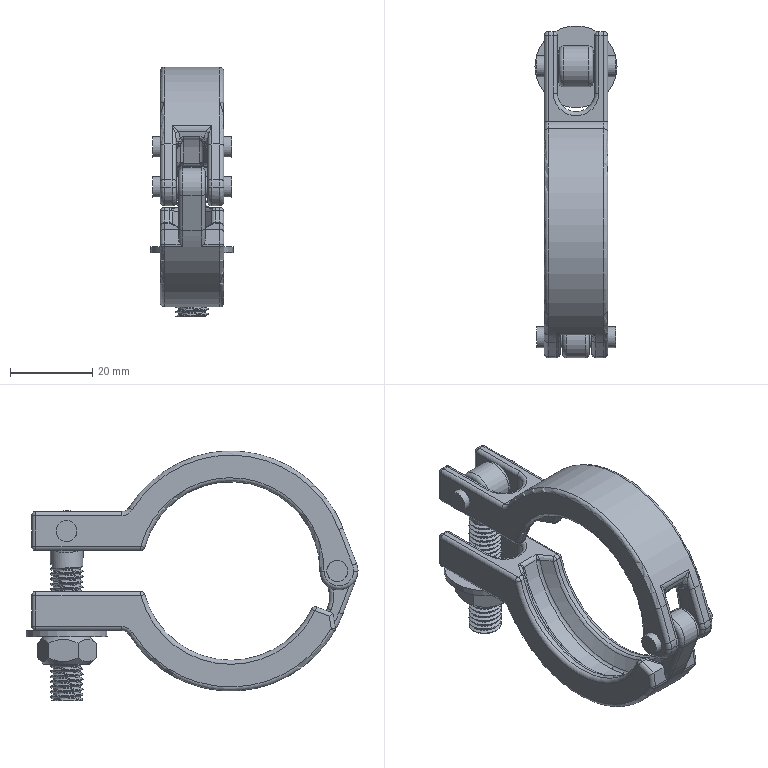Assembly | NX | mm | 7 component files | 7 solids | 308 faces | box 20 x 81 x 60.9 mm | volume 18749 mm3 | cylinder 119 | torus 52 | spline 48 | plane 47 | sphere 34 | cone 8 | commonest cylinder face diameters 2 x57 7.94 x26 5.1 x8 43.5 x4 4 x3 10 x3 8 x2 58.5 x2
Bill of materials:
unnamed part 1 | 1 |  | Hexagonal nut with a central threaded through-bore and chamfered corners on both faces.
unnamed part 2 | 1 |  | Eye bolt: a straight threaded shank with a short plain neck, ending in a round eye whose through-hole runs perpendicular to the shank axis.
unnamed part 3 | 2 |  | Plain solid cylinder (round rod or pin) with flat ends.
unnamed part 4 | 1 |  | Flat washer: a thin circular disc with a concentric through-hole.
unnamed part 5 | 1 |  | Curved clamp or strap segment: a semicircular-ish arc band that joins a straight offset arm. Both ends are forked into two parallel prongs, and each prong has a cross hole.
unnamed part 6 | 1 |  | Curved clamp or strap segment: an arc band with a concave inner channel, a single centred eye tab with a hole at the curved end, and a straight arm forked into two prongs at the other end.
Mates:
1. fix | upper_clasp 1 component
2. align lock | pin 1 face | upper_clasp 1 face
3. distance | pin 1 face | upper_clasp 1 face
4. align lock | bolt 1 face | pin 1 face
5. distance | bolt 1 face | upper_clasp 1 face
6. align lock | pin 2 face | upper_clasp 1 face
7. distance | pin 2 face | upper_clasp 1 face
8. align lock | lower_clasp 1 face | pin 2 face
9. distance | lower_clasp 1 face | upper_clasp 1 face
10. concentric | nut 1 edge | washer 1 edge
11. align lock | nut 1 face | bolt 1 face
12. touch align | washer 1 face | lower_clasp 1 face